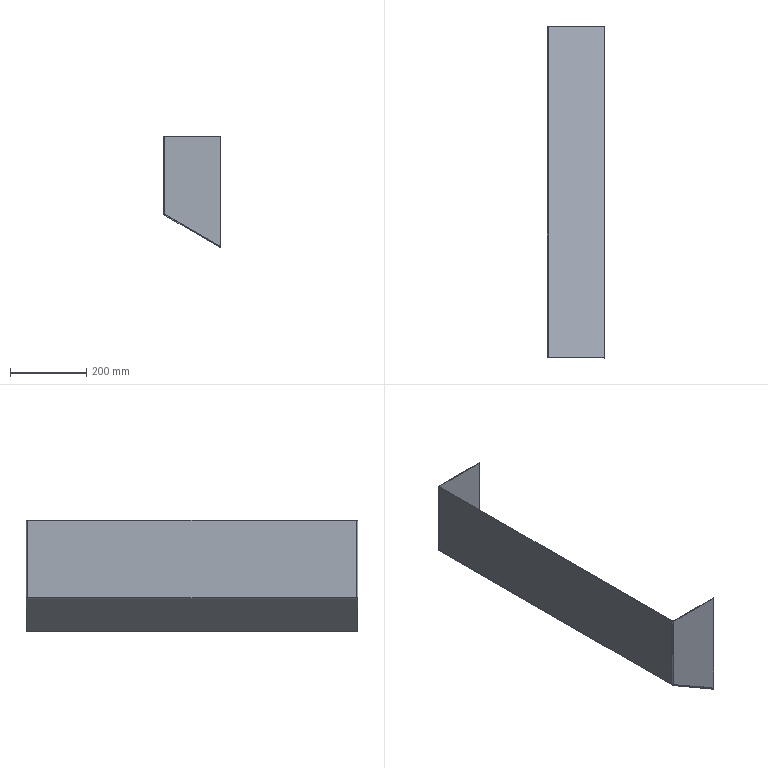Component | SolidWorks | AirInletUpperBeamAssembly-1_AirInletUpperBeamBaffle-2 | 1 solid | 32 faces | box 152 x 870 x 291.73 mm | volume 803027 mm3 | plane 24 | cylinder 6 | spline 2 | commonest cylinder face diameters 4 x3 8 x3 | material Plain Carbon Steel
STEP:
#1=COLOUR_RGB('',0.7922,0.8196,0.9333);
#2=FILL_AREA_STYLE_COLOUR('',#1);
#3=FILL_AREA_STYLE('',(#2));
#4=SURFACE_STYLE_FILL_AREA(#3);
#5=SURFACE_SIDE_STYLE('',(#4));
#6=SURFACE_STYLE_USAGE(.BOTH.,#5);
#7=PRESENTATION_STYLE_ASSIGNMENT((#6));
#8=CARTESIAN_POINT('',(95.562,7.226,69.616));
#9=VERTEX_POINT('',#8);
#10=CARTESIAN_POINT('',(95.562,41.163,69.616));
#11=VERTEX_POINT('',#10);
#12=CARTESIAN_POINT('',(95.562,7.069,69.616));
#13=DIRECTION('',(-0.,1.,-0.));
#14=VECTOR('',#13,39.37);
#15=LINE('',#12,#14);
#16=EDGE_CURVE('',#9,#11,#15,.T.);
#17=ORIENTED_EDGE('',*,*,#16,.T.);
#18=CARTESIAN_POINT('',(95.562,41.163,77.578));
#19=VERTEX_POINT('',#18);
#20=CARTESIAN_POINT('',(95.562,41.163,77.578));
#21=DIRECTION('',(0.,-0.,-1.));
#22=VECTOR('',#21,39.37);
#23=LINE('',#20,#22);
#24=EDGE_CURVE('',#19,#11,#23,.T.);
#25=ORIENTED_EDGE('',*,*,#24,.F.);
#26=CARTESIAN_POINT('',(95.562,7.226,77.578));
#27=VERTEX_POINT('',#26);
#28=CARTESIAN_POINT('',(95.562,7.069,77.578));
#29=DIRECTION('',(-0.,1.,-0.));
#30=VECTOR('',#29,39.37);
#31=LINE('',#28,#30);
#32=EDGE_CURVE('',#27,#19,#31,.T.);
#33=ORIENTED_EDGE('',*,*,#32,.F.);
#34=CARTESIAN_POINT('',(95.562,7.226,69.57));
#35=DIRECTION('',(-0.,0.,1.));
#36=VECTOR('',#35,39.37);
#37=LINE('',#34,#36);
#38=EDGE_CURVE('',#9,#27,#37,.T.);
#39=ORIENTED_EDGE('',*,*,#38,.F.);
#40=EDGE_LOOP('',(#17,#25,#33,#39));
#41=FACE_OUTER_BOUND('',#40,.T.);
#42=CARTESIAN_POINT('',(95.562,7.069,69.57));
#43=DIRECTION('',(1.,0.,-0.));
#44=DIRECTION('',(0.,0.,1.));
#45=AXIS2_PLACEMENT_3D('',#42,#43,#44);
#46=PLANE('',#45);
#47=ADVANCED_FACE('',(#41),#46,.T.);
#48=CARTESIAN_POINT('',(95.484,41.163,77.578));
#49=VERTEX_POINT('',#48);
#50=CARTESIAN_POINT('',(95.484,41.163,69.616));
#51=VERTEX_POINT('',#50);
#52=CARTESIAN_POINT('',(95.484,41.163,77.578));
#53=DIRECTION('',(0.,-0.,-1.));
#54=VECTOR('',#53,39.37);
#55=LINE('',#52,#54);
#56=EDGE_CURVE('',#49,#51,#55,.T.);
#57=ORIENTED_EDGE('',*,*,#56,.T.);
#58=CARTESIAN_POINT('',(95.484,7.226,69.616));
#59=VERTEX_POINT('',#58);
#60=CARTESIAN_POINT('',(95.484,7.069,69.616));
#61=DIRECTION('',(-0.,1.,-0.));
#62=VECTOR('',#61,39.37);
#63=LINE('',#60,#62);
#64=EDGE_CURVE('',#59,#51,#63,.T.);
#65=ORIENTED_EDGE('',*,*,#64,.F.);
#66=CARTESIAN_POINT('',(95.484,7.226,77.578));
#67=VERTEX_POINT('',#66);
#68=CARTESIAN_POINT('',(95.484,7.226,69.57));
#69=DIRECTION('',(-0.,0.,1.));
#70=VECTOR('',#69,39.37);
#71=LINE('',#68,#70);
#72=EDGE_CURVE('',#59,#67,#71,.T.);
#73=ORIENTED_EDGE('',*,*,#72,.T.);
#74=CARTESIAN_POINT('',(95.484,7.069,77.578));
#75=DIRECTION('',(-0.,1.,-0.));
#76=VECTOR('',#75,39.37);
#77=LINE('',#74,#76);
#78=EDGE_CURVE('',#67,#49,#77,.T.);
#79=ORIENTED_EDGE('',*,*,#78,.T.);
#80=EDGE_LOOP('',(#57,#65,#73,#79));
#81=FACE_OUTER_BOUND('',#80,.T.);
#82=CARTESIAN_POINT('',(95.484,7.069,69.57));
#83=DIRECTION('',(1.,0.,-0.));
#84=DIRECTION('',(0.,0.,1.));
#85=AXIS2_PLACEMENT_3D('',#82,#83,#84);
#86=PLANE('',#85);
#87=ADVANCED_FACE('',(#81),#86,.F.);
#88=ORIENTED_EDGE('',*,*,#32,.T.);
#89=CARTESIAN_POINT('',(95.562,41.163,77.578));
#90=DIRECTION('',(-1.,-0.,0.));
#91=VECTOR('',#90,39.37);
#92=LINE('',#89,#91);
#93=EDGE_CURVE('',#19,#49,#92,.T.);
#94=ORIENTED_EDGE('',*,*,#93,.T.);
#95=ORIENTED_EDGE('',*,*,#78,.F.);
#96=CARTESIAN_POINT('',(95.562,7.226,77.578));
#97=DIRECTION('',(-1.,-0.,0.));
#98=VECTOR('',#97,39.37);
#99=LINE('',#96,#98);
#100=EDGE_CURVE('',#27,#67,#99,.T.);
#101=ORIENTED_EDGE('',*,*,#100,.F.);
#102=EDGE_LOOP('',(#88,#94,#95,#101));
#103=FACE_OUTER_BOUND('',#102,.T.);
#104=CARTESIAN_POINT('',(95.484,7.069,77.578));
#105=DIRECTION('',(-0.,0.,1.));
#106=DIRECTION('',(0.,-1.,0.));
#107=AXIS2_PLACEMENT_3D('',#104,#105,#106);
#108=PLANE('',#107);
#109=ADVANCED_FACE('',(#103),#108,.T.);
#110=CARTESIAN_POINT('',(95.602,7.069,69.547));
#111=VERTEX_POINT('',#110);
#112=CARTESIAN_POINT('',(95.562,7.069,69.479));
#113=VERTEX_POINT('',#112);
#114=CARTESIAN_POINT('',(95.602,7.069,69.547));
#115=DIRECTION('',(-0.5,-0.,-0.866));
#116=VECTOR('',#115,39.37);
#117=LINE('',#114,#116);
#118=EDGE_CURVE('',#111,#113,#117,.T.);
#119=ORIENTED_EDGE('',*,*,#118,.F.);
#120=CARTESIAN_POINT('',(95.562,7.069,69.616));
#121=VERTEX_POINT('',#120);
#122=CARTESIAN_POINT('',(95.641,7.069,69.616));
#123=DIRECTION('',(0.,-1.,0.));
#124=DIRECTION('',(-1.,0.,0.));
#125=AXIS2_PLACEMENT_3D('',#122,#123,#124);
#126=CIRCLE('',#125,0.07874);
#127=EDGE_CURVE('',#121,#111,#126,.T.);
#128=ORIENTED_EDGE('',*,*,#127,.F.);
#129=CARTESIAN_POINT('',(95.484,7.069,69.616));
#130=VERTEX_POINT('',#129);
#131=CARTESIAN_POINT('',(95.484,7.069,69.616));
#132=DIRECTION('',(1.,0.,-0.));
#133=VECTOR('',#132,39.37);
#134=LINE('',#131,#133);
#135=EDGE_CURVE('',#130,#121,#134,.T.);
#136=ORIENTED_EDGE('',*,*,#135,.F.);
#137=CARTESIAN_POINT('',(95.641,7.069,69.616));
#138=DIRECTION('',(0.,-1.,0.));
#139=DIRECTION('',(1.,0.,0.));
#140=AXIS2_PLACEMENT_3D('',#137,#138,#139);
#141=CIRCLE('',#140,0.1575);
#142=EDGE_CURVE('',#130,#113,#141,.T.);
#143=ORIENTED_EDGE('',*,*,#142,.T.);
#144=EDGE_LOOP('',(#119,#128,#136,#143));
#145=FACE_OUTER_BOUND('',#144,.T.);
#146=CARTESIAN_POINT('',(95.602,7.069,69.547));
#147=DIRECTION('',(0.,-1.,0.));
#148=DIRECTION('',(1.,0.,-0.));
#149=AXIS2_PLACEMENT_3D('',#146,#147,#148);
#150=PLANE('',#149);
#151=ADVANCED_FACE('',(#145),#150,.T.);
#152=CARTESIAN_POINT('',(101.468,7.069,66.161));
#153=VERTEX_POINT('',#152);
#154=CARTESIAN_POINT('',(95.562,7.069,69.57));
#155=DIRECTION('',(0.866,0.,-0.5));
#156=VECTOR('',#155,39.37);
#157=LINE('',#154,#156);
#158=EDGE_CURVE('',#111,#153,#157,.T.);
#159=ORIENTED_EDGE('',*,*,#158,.F.);
#160=ORIENTED_EDGE('',*,*,#118,.T.);
#161=CARTESIAN_POINT('',(101.429,7.069,66.092));
#162=VERTEX_POINT('',#161);
#163=CARTESIAN_POINT('',(95.523,7.069,69.502));
#164=DIRECTION('',(0.866,0.,-0.5));
#165=VECTOR('',#164,39.37);
#166=LINE('',#163,#165);
#167=EDGE_CURVE('',#113,#162,#166,.T.);
#168=ORIENTED_EDGE('',*,*,#167,.T.);
#169=CARTESIAN_POINT('',(101.468,7.069,66.161));
#170=DIRECTION('',(-0.5,-0.,-0.866));
#171=VECTOR('',#170,39.37);
#172=LINE('',#169,#171);
#173=EDGE_CURVE('',#153,#162,#172,.T.);
#174=ORIENTED_EDGE('',*,*,#173,.F.);
#175=EDGE_LOOP('',(#159,#160,#168,#174));
#176=FACE_OUTER_BOUND('',#175,.T.);
#177=CARTESIAN_POINT('',(95.484,7.069,69.616));
#178=DIRECTION('',(0.,-1.,0.));
#179=DIRECTION('',(1.,0.,-0.));
#180=AXIS2_PLACEMENT_3D('',#177,#178,#179);
#181=PLANE('',#180);
#182=ADVANCED_FACE('',(#176),#181,.T.);
#183=CARTESIAN_POINT('',(95.562,41.321,69.616));
#184=VERTEX_POINT('',#183);
#185=CARTESIAN_POINT('',(95.484,41.321,69.616));
#186=VERTEX_POINT('',#185);
#187=CARTESIAN_POINT('',(95.562,41.321,69.616));
#188=DIRECTION('',(-1.,-0.,0.));
#189=VECTOR('',#188,39.37);
#190=LINE('',#187,#189);
#191=EDGE_CURVE('',#184,#186,#190,.T.);
#192=ORIENTED_EDGE('',*,*,#191,.F.);
#193=CARTESIAN_POINT('',(95.602,41.321,69.547));
#194=VERTEX_POINT('',#193);
#195=CARTESIAN_POINT('',(95.641,41.321,69.616));
#196=DIRECTION('',(0.,-1.,0.));
#197=DIRECTION('',(-1.,0.,0.));
#198=AXIS2_PLACEMENT_3D('',#195,#196,#197);
#199=CIRCLE('',#198,0.07874);
#200=EDGE_CURVE('',#184,#194,#199,.T.);
#201=ORIENTED_EDGE('',*,*,#200,.T.);
#202=CARTESIAN_POINT('',(95.562,41.321,69.479));
#203=VERTEX_POINT('',#202);
#204=CARTESIAN_POINT('',(95.562,41.321,69.479));
#205=DIRECTION('',(0.5,0.,0.866));
#206=VECTOR('',#205,39.37);
#207=LINE('',#204,#206);
#208=EDGE_CURVE('',#203,#194,#207,.T.);
#209=ORIENTED_EDGE('',*,*,#208,.F.);
#210=CARTESIAN_POINT('',(95.641,41.321,69.616));
#211=DIRECTION('',(0.,-1.,0.));
#212=DIRECTION('',(1.,0.,0.));
#213=AXIS2_PLACEMENT_3D('',#210,#211,#212);
#214=CIRCLE('',#213,0.1575);
#215=EDGE_CURVE('',#186,#203,#214,.T.);
#216=ORIENTED_EDGE('',*,*,#215,.F.);
#217=EDGE_LOOP('',(#192,#201,#209,#216));
#218=FACE_OUTER_BOUND('',#217,.T.);
#219=CARTESIAN_POINT('',(95.562,41.321,69.616));
#220=DIRECTION('',(-0.,1.,-0.));
#221=DIRECTION('',(-1.,-0.,0.));
#222=AXIS2_PLACEMENT_3D('',#219,#220,#221);
#223=PLANE('',#222);
#224=ADVANCED_FACE('',(#218),#223,.T.);
#225=CARTESIAN_POINT('',(101.429,41.321,66.092));
#226=VERTEX_POINT('',#225);
#227=CARTESIAN_POINT('',(95.523,41.321,69.502));
#228=DIRECTION('',(0.866,0.,-0.5));
#229=VECTOR('',#228,39.37);
#230=LINE('',#227,#229);
#231=EDGE_CURVE('',#203,#226,#230,.T.);
#232=ORIENTED_EDGE('',*,*,#231,.T.);
#233=CARTESIAN_POINT('',(101.429,7.069,66.092));
#234=DIRECTION('',(-0.,1.,-0.));
#235=VECTOR('',#234,39.37);
#236=LINE('',#233,#235);
#237=EDGE_CURVE('',#162,#226,#236,.T.);
#238=ORIENTED_EDGE('',*,*,#237,.F.);
#239=ORIENTED_EDGE('',*,*,#167,.F.);
#240=CARTESIAN_POINT('',(95.562,7.069,69.479));
#241=DIRECTION('',(-0.,1.,-0.));
#242=VECTOR('',#241,39.37);
#243=LINE('',#240,#242);
#244=EDGE_CURVE('',#113,#203,#243,.T.);
#245=ORIENTED_EDGE('',*,*,#244,.T.);
#246=EDGE_LOOP('',(#232,#238,#239,#245));
#247=FACE_OUTER_BOUND('',#246,.T.);
#248=CARTESIAN_POINT('',(95.523,7.069,69.502));
#249=DIRECTION('',(0.5,0.,0.866));
#250=DIRECTION('',(-0.866,-0.,0.5));
#251=AXIS2_PLACEMENT_3D('',#248,#249,#250);
#252=PLANE('',#251);
#253=ADVANCED_FACE('',(#247),#252,.F.);
#254=CARTESIAN_POINT('',(101.468,41.321,66.161));
#255=VERTEX_POINT('',#254);
#256=CARTESIAN_POINT('',(101.468,41.321,66.161));
#257=DIRECTION('',(-0.5,-0.,-0.866));
#258=VECTOR('',#257,39.37);
#259=LINE('',#256,#258);
#260=EDGE_CURVE('',#255,#226,#259,.T.);
#261=ORIENTED_EDGE('',*,*,#260,.F.);
#262=CARTESIAN_POINT('',(101.468,7.069,66.161));
#263=DIRECTION('',(-0.,1.,-0.));
#264=VECTOR('',#263,39.37);
#265=LINE('',#262,#264);
#266=EDGE_CURVE('',#153,#255,#265,.T.);
#267=ORIENTED_EDGE('',*,*,#266,.F.);
#268=ORIENTED_EDGE('',*,*,#173,.T.);
#269=ORIENTED_EDGE('',*,*,#237,.T.);
#270=EDGE_LOOP('',(#261,#267,#268,#269));
#271=FACE_OUTER_BOUND('',#270,.T.);
#272=CARTESIAN_POINT('',(101.468,7.069,66.161));
#273=DIRECTION('',(0.866,0.,-0.5));
#274=DIRECTION('',(0.5,0.,0.866));
#275=AXIS2_PLACEMENT_3D('',#272,#273,#274);
#276=PLANE('',#275);
#277=ADVANCED_FACE('',(#271),#276,.T.);
#278=CARTESIAN_POINT('',(95.562,41.321,69.57));
#279=DIRECTION('',(0.866,0.,-0.5));
#280=VECTOR('',#279,39.37);
#281=LINE('',#278,#280);
#282=EDGE_CURVE('',#194,#255,#281,.T.);
#283=ORIENTED_EDGE('',*,*,#282,.F.);
#284=CARTESIAN_POINT('',(95.602,7.069,69.547));
#285=DIRECTION('',(-0.,1.,-0.));
#286=VECTOR('',#285,39.37);
#287=LINE('',#284,#286);
#288=EDGE_CURVE('',#111,#194,#287,.T.);
#289=ORIENTED_EDGE('',*,*,#288,.F.);
#290=ORIENTED_EDGE('',*,*,#158,.T.);
#291=ORIENTED_EDGE('',*,*,#266,.T.);
#292=EDGE_LOOP('',(#283,#289,#290,#291));
#293=FACE_OUTER_BOUND('',#292,.T.);
#294=CARTESIAN_POINT('',(95.562,7.069,69.57));
#295=DIRECTION('',(0.5,0.,0.866));
#296=DIRECTION('',(-0.866,-0.,0.5));
#297=AXIS2_PLACEMENT_3D('',#294,#295,#296);
#298=PLANE('',#297);
#299=ADVANCED_FACE('',(#293),#298,.T.);
#300=ORIENTED_EDGE('',*,*,#200,.F.);
#301=CARTESIAN_POINT('',(95.562,41.163,69.616));
#302=DIRECTION('',(-0.,1.,0.));
#303=VECTOR('',#302,39.37);
#304=LINE('',#301,#303);
#305=EDGE_CURVE('',#11,#184,#304,.T.);
#306=ORIENTED_EDGE('',*,*,#305,.F.);
#307=ORIENTED_EDGE('',*,*,#16,.F.);
#308=CARTESIAN_POINT('',(95.562,7.069,69.616));
#309=DIRECTION('',(-0.,1.,-0.));
#310=VECTOR('',#309,39.37);
#311=LINE('',#308,#310);
#312=EDGE_CURVE('',#121,#9,#311,.T.);
#313=ORIENTED_EDGE('',*,*,#312,.F.);
#314=ORIENTED_EDGE('',*,*,#127,.T.);
#315=ORIENTED_EDGE('',*,*,#288,.T.);
#316=EDGE_LOOP('',(#300,#306,#307,#313,#314,#315));
#317=FACE_OUTER_BOUND('',#316,.T.);
#318=CARTESIAN_POINT('',(95.641,7.069,69.616));
#319=DIRECTION('',(-0.,1.,-0.));
#320=DIRECTION('',(-1.,0.,0.));
#321=AXIS2_PLACEMENT_3D('',#318,#319,#320);
#322=CYLINDRICAL_SURFACE('',#321,0.07874);
#323=ADVANCED_FACE('',(#317),#322,.F.);
#324=ORIENTED_EDGE('',*,*,#215,.T.);
#325=ORIENTED_EDGE('',*,*,#244,.F.);
#326=ORIENTED_EDGE('',*,*,#142,.F.);
#327=CARTESIAN_POINT('',(95.484,7.069,69.616));
#328=DIRECTION('',(-0.,1.,-0.));
#329=VECTOR('',#328,39.37);
#330=LINE('',#327,#329);
#331=EDGE_CURVE('',#130,#59,#330,.T.);
#332=ORIENTED_EDGE('',*,*,#331,.T.);
#333=ORIENTED_EDGE('',*,*,#64,.T.);
#334=CARTESIAN_POINT('',(95.484,7.069,69.616));
#335=DIRECTION('',(-0.,1.,-0.));
#336=VECTOR('',#335,39.37);
#337=LINE('',#334,#336);
#338=EDGE_CURVE('',#51,#186,#337,.T.);
#339=ORIENTED_EDGE('',*,*,#338,.T.);
#340=EDGE_LOOP('',(#324,#325,#326,#332,#333,#339));
#341=FACE_OUTER_BOUND('',#340,.T.);
#342=CARTESIAN_POINT('',(95.641,7.069,69.616));
#343=DIRECTION('',(-0.,1.,-0.));
#344=DIRECTION('',(-1.,-0.,0.));
#345=AXIS2_PLACEMENT_3D('',#342,#343,#344);
#346=CYLINDRICAL_SURFACE('',#345,0.1575);
#347=ADVANCED_FACE('',(#341),#346,.T.);
#348=ORIENTED_EDGE('',*,*,#231,.F.);
#349=ORIENTED_EDGE('',*,*,#208,.T.);
#350=ORIENTED_EDGE('',*,*,#282,.T.);
#351=ORIENTED_EDGE('',*,*,#260,.T.);
#352=EDGE_LOOP('',(#348,#349,#350,#351));
#353=FACE_OUTER_BOUND('',#352,.T.);
#354=CARTESIAN_POINT('',(95.641,41.321,69.616));
#355=DIRECTION('',(-0.,1.,-0.));
#356=DIRECTION('',(-1.,-0.,0.));
#357=AXIS2_PLACEMENT_3D('',#354,#355,#356);
#358=PLANE('',#357);
#359=ADVANCED_FACE('',(#353),#358,.T.);
#360=CARTESIAN_POINT('',(95.562,7.226,69.616));
#361=DIRECTION('',(-1.,-0.,0.));
#362=VECTOR('',#361,39.37);
#363=LINE('',#360,#362);
#364=EDGE_CURVE('',#9,#59,#363,.T.);
#365=ORIENTED_EDGE('',*,*,#364,.T.);
#366=ORIENTED_EDGE('',*,*,#331,.F.);
#367=ORIENTED_EDGE('',*,*,#135,.T.);
#368=ORIENTED_EDGE('',*,*,#312,.T.);
#369=EDGE_LOOP('',(#365,#366,#367,#368));
#370=FACE_OUTER_BOUND('',#369,.T.);
#371=CARTESIAN_POINT('',(95.562,7.069,69.616));
#372=DIRECTION('',(0.,0.,1.));
#373=DIRECTION('',(0.,-1.,0.));
#374=AXIS2_PLACEMENT_3D('',#371,#372,#373);
#375=PLANE('',#374);
#376=ADVANCED_FACE('',(#370),#375,.T.);
#377=CARTESIAN_POINT('',(95.641,7.148,77.578));
#378=VERTEX_POINT('',#377);
#379=CARTESIAN_POINT('',(95.641,7.069,77.578));
#380=VERTEX_POINT('',#379);
#381=CARTESIAN_POINT('',(95.641,7.069,77.578));
#382=DIRECTION('',(0.,-1.,0.));
#383=VECTOR('',#382,39.37);
#384=LINE('',#381,#383);
#385=EDGE_CURVE('',#378,#380,#384,.T.);
#386=ORIENTED_EDGE('',*,*,#385,.F.);
#387=CARTESIAN_POINT('',(95.641,7.226,77.578));
#388=DIRECTION('',(-0.,0.,1.));
#389=DIRECTION('',(0.,1.,0.));
#390=AXIS2_PLACEMENT_3D('',#387,#388,#389);
#391=CIRCLE('',#390,0.07874);
#392=EDGE_CURVE('',#27,#378,#391,.T.);
#393=ORIENTED_EDGE('',*,*,#392,.F.);
#394=ORIENTED_EDGE('',*,*,#100,.T.);
#395=CARTESIAN_POINT('',(95.641,7.226,77.578));
#396=DIRECTION('',(-0.,0.,1.));
#397=DIRECTION('',(0.,1.,0.));
#398=AXIS2_PLACEMENT_3D('',#395,#396,#397);
#399=CIRCLE('',#398,0.1575);
#400=EDGE_CURVE('',#67,#380,#399,.T.);
#401=ORIENTED_EDGE('',*,*,#400,.T.);
#402=EDGE_LOOP('',(#386,#393,#394,#401));
#403=FACE_OUTER_BOUND('',#402,.T.);
#404=CARTESIAN_POINT('',(95.641,7.226,77.578));
#405=DIRECTION('',(-0.,0.,1.));
#406=DIRECTION('',(0.,-1.,0.));
#407=AXIS2_PLACEMENT_3D('',#404,#405,#406);
#408=PLANE('',#407);
#409=ADVANCED_FACE('',(#403),#408,.T.);
#410=CARTESIAN_POINT('',(95.641,7.148,69.57));
#411=VERTEX_POINT('',#410);
#412=CARTESIAN_POINT('',(95.641,7.148,69.57));
#413=CARTESIAN_POINT('',(95.636,7.148,69.572));
#414=CARTESIAN_POINT('',(95.631,7.148,69.574));
#415=CARTESIAN_POINT('',(95.621,7.15,69.578));
#416=CARTESIAN_POINT('',(95.616,7.152,69.58));
#417=CARTESIAN_POINT('',(95.606,7.156,69.583));
#418=CARTESIAN_POINT('',(95.602,7.158,69.585));
#419=CARTESIAN_POINT('',(95.593,7.164,69.589));
#420=CARTESIAN_POINT('',(95.589,7.167,69.591));
#421=CARTESIAN_POINT('',(95.582,7.174,69.595));
#422=CARTESIAN_POINT('',(95.579,7.178,69.597));
#423=CARTESIAN_POINT('',(95.573,7.187,69.6));
#424=CARTESIAN_POINT('',(95.57,7.191,69.602));
#425=CARTESIAN_POINT('',(95.567,7.201,69.606));
#426=CARTESIAN_POINT('',(95.565,7.206,69.608));
#427=CARTESIAN_POINT('',(95.563,7.216,69.612));
#428=CARTESIAN_POINT('',(95.562,7.221,69.614));
#429=CARTESIAN_POINT('',(95.562,7.226,69.616));
#430=B_SPLINE_CURVE_WITH_KNOTS('',3,(#412,#413,#414,#415,#416,#417,#418,#419,#420,#421,#422,#423,#424,#425,#426,#427,#428,#429),.UNSPECIFIED.,.F.,.F.,(4,2,2,2,2,2,2,2,4),(0.,0.0004161,0.0008322,0.001248,0.001664,0.002081,0.002497,0.002913,0.003329),.UNSPECIFIED.);
#431=EDGE_CURVE('',#411,#9,#430,.T.);
#432=ORIENTED_EDGE('',*,*,#431,.F.);
#433=CARTESIAN_POINT('',(95.641,7.069,69.57));
#434=VERTEX_POINT('',#433);
#435=CARTESIAN_POINT('',(95.641,7.148,69.57));
#436=DIRECTION('',(0.,-1.,-0.));
#437=VECTOR('',#436,39.37);
#438=LINE('',#435,#437);
#439=EDGE_CURVE('',#411,#434,#438,.T.);
#440=ORIENTED_EDGE('',*,*,#439,.T.);
#441=CARTESIAN_POINT('',(95.641,7.069,69.57));
#442=CARTESIAN_POINT('',(95.631,7.069,69.572));
#443=CARTESIAN_POINT('',(95.621,7.07,69.574));
#444=CARTESIAN_POINT('',(95.6,7.074,69.578));
#445=CARTESIAN_POINT('',(95.59,7.077,69.58));
#446=CARTESIAN_POINT('',(95.571,7.085,69.583));
#447=CARTESIAN_POINT('',(95.562,7.09,69.585));
#448=CARTESIAN_POINT('',(95.545,7.101,69.589));
#449=CARTESIAN_POINT('',(95.537,7.108,69.591));
#450=CARTESIAN_POINT('',(95.523,7.122,69.595));
#451=CARTESIAN_POINT('',(95.516,7.13,69.597));
#452=CARTESIAN_POINT('',(95.505,7.147,69.6));
#453=CARTESIAN_POINT('',(95.5,7.156,69.602));
#454=CARTESIAN_POINT('',(95.488,7.185,69.608));
#455=CARTESIAN_POINT('',(95.484,7.206,69.612));
#456=CARTESIAN_POINT('',(95.484,7.226,69.616));
#457=B_SPLINE_CURVE_WITH_KNOTS('',3,(#441,#442,#443,#444,#445,#446,#447,#448,#449,#450,#451,#452,#453,#454,#455,#456),.UNSPECIFIED.,.F.,.F.,(4,2,2,2,2,2,2,4),(0.,0.0007941,0.001588,0.002382,0.003177,0.003971,0.004765,0.006353),.UNSPECIFIED.);
#458=EDGE_CURVE('',#434,#59,#457,.T.);
#459=ORIENTED_EDGE('',*,*,#458,.T.);
#460=ORIENTED_EDGE('',*,*,#364,.F.);
#461=EDGE_LOOP('',(#432,#440,#459,#460));
#462=FACE_OUTER_BOUND('',#461,.T.);
#463=CARTESIAN_POINT('',(95.641,7.068,69.57));
#464=CARTESIAN_POINT('',(95.62,7.068,69.574));
#465=CARTESIAN_POINT('',(95.6,7.072,69.578));
#466=CARTESIAN_POINT('',(95.562,7.088,69.585));
#467=CARTESIAN_POINT('',(95.544,7.1,69.589));
#468=CARTESIAN_POINT('',(95.515,7.129,69.597));
#469=CARTESIAN_POINT('',(95.503,7.147,69.6));
#470=CARTESIAN_POINT('',(95.487,7.185,69.608));
#471=CARTESIAN_POINT('',(95.483,7.206,69.612));
#472=CARTESIAN_POINT('',(95.483,7.226,69.616));
#473=CARTESIAN_POINT('',(95.641,7.069,69.57));
#474=CARTESIAN_POINT('',(95.621,7.069,69.574));
#475=CARTESIAN_POINT('',(95.6,7.073,69.578));
#476=CARTESIAN_POINT('',(95.562,7.089,69.585));
#477=CARTESIAN_POINT('',(95.544,7.1,69.589));
#478=CARTESIAN_POINT('',(95.515,7.13,69.597));
#479=CARTESIAN_POINT('',(95.504,7.147,69.6));
#480=CARTESIAN_POINT('',(95.488,7.185,69.608));
#481=CARTESIAN_POINT('',(95.484,7.206,69.612));
#482=CARTESIAN_POINT('',(95.484,7.226,69.616));
#483=CARTESIAN_POINT('',(95.641,7.148,69.57));
#484=CARTESIAN_POINT('',(95.631,7.148,69.574));
#485=CARTESIAN_POINT('',(95.621,7.15,69.578));
#486=CARTESIAN_POINT('',(95.602,7.158,69.585));
#487=CARTESIAN_POINT('',(95.593,7.163,69.589));
#488=CARTESIAN_POINT('',(95.578,7.178,69.597));
#489=CARTESIAN_POINT('',(95.572,7.187,69.6));
#490=CARTESIAN_POINT('',(95.565,7.206,69.608));
#491=CARTESIAN_POINT('',(95.562,7.216,69.612));
#492=CARTESIAN_POINT('',(95.562,7.226,69.616));
#493=CARTESIAN_POINT('',(95.641,7.148,69.57));
#494=CARTESIAN_POINT('',(95.631,7.148,69.574));
#495=CARTESIAN_POINT('',(95.621,7.15,69.578));
#496=CARTESIAN_POINT('',(95.602,7.158,69.585));
#497=CARTESIAN_POINT('',(95.593,7.164,69.589));
#498=CARTESIAN_POINT('',(95.579,7.178,69.597));
#499=CARTESIAN_POINT('',(95.573,7.187,69.6));
#500=CARTESIAN_POINT('',(95.565,7.206,69.608));
#501=CARTESIAN_POINT('',(95.563,7.216,69.612));
#502=CARTESIAN_POINT('',(95.563,7.226,69.616));
#503=B_SPLINE_SURFACE_WITH_KNOTS('',1,3,((#463,#464,#465,#466,#467,#468,#469,#470,#471,#472),(#473,#474,#475,#476,#477,#478,#479,#480,#481,#482),(#483,#484,#485,#486,#487,#488,#489,#490,#491,#492),(#493,#494,#495,#496,#497,#498,#499,#500,#501,#502)),.UNSPECIFIED.,.F.,.F.,.F.,(2,1,1,2),(4,2,2,2,4),(-0.01,0.,1.,1.01),(0.,0.25,0.5,0.75,1.),.UNSPECIFIED.);
#504=ADVANCED_FACE('',(#462),#503,.F.);
#505=ORIENTED_EDGE('',*,*,#72,.F.);
#506=ORIENTED_EDGE('',*,*,#458,.F.);
#507=CARTESIAN_POINT('',(95.641,7.069,77.578));
#508=DIRECTION('',(-0.,0.,1.));
#509=VECTOR('',#508,39.37);
#510=LINE('',#507,#509);
#511=EDGE_CURVE('',#434,#380,#510,.T.);
#512=ORIENTED_EDGE('',*,*,#511,.T.);
#513=ORIENTED_EDGE('',*,*,#400,.F.);
#514=EDGE_LOOP('',(#505,#506,#512,#513));
#515=FACE_OUTER_BOUND('',#514,.T.);
#516=CARTESIAN_POINT('',(95.641,7.226,69.57));
#517=DIRECTION('',(0.,-0.,-1.));
#518=DIRECTION('',(0.,-1.,0.));
#519=AXIS2_PLACEMENT_3D('',#516,#517,#518);
#520=CYLINDRICAL_SURFACE('',#519,0.1575);
#521=ADVANCED_FACE('',(#515),#520,.T.);
#522=ORIENTED_EDGE('',*,*,#38,.T.);
#523=ORIENTED_EDGE('',*,*,#392,.T.);
#524=CARTESIAN_POINT('',(95.641,7.148,77.578));
#525=DIRECTION('',(0.,-0.,-1.));
#526=VECTOR('',#525,39.37);
#527=LINE('',#524,#526);
#528=EDGE_CURVE('',#378,#411,#527,.T.);
#529=ORIENTED_EDGE('',*,*,#528,.T.);
#530=ORIENTED_EDGE('',*,*,#431,.T.);
#531=EDGE_LOOP('',(#522,#523,#529,#530));
#532=FACE_OUTER_BOUND('',#531,.T.);
#533=CARTESIAN_POINT('',(95.641,7.226,69.57));
#534=DIRECTION('',(0.,-0.,-1.));
#535=DIRECTION('',(0.,-1.,0.));
#536=AXIS2_PLACEMENT_3D('',#533,#534,#535);
#537=CYLINDRICAL_SURFACE('',#536,0.07874);
#538=ADVANCED_FACE('',(#532),#537,.F.);
#539=ORIENTED_EDGE('',*,*,#385,.T.);
#540=CARTESIAN_POINT('',(101.468,7.069,77.578));
#541=VERTEX_POINT('',#540);
#542=CARTESIAN_POINT('',(95.562,7.069,77.578));
#543=DIRECTION('',(-1.,0.,0.));
#544=VECTOR('',#543,39.37);
#545=LINE('',#542,#544);
#546=EDGE_CURVE('',#541,#380,#545,.T.);
#547=ORIENTED_EDGE('',*,*,#546,.F.);
#548=CARTESIAN_POINT('',(101.468,7.148,77.578));
#549=VERTEX_POINT('',#548);
#550=CARTESIAN_POINT('',(101.468,7.069,77.578));
#551=DIRECTION('',(-0.,1.,-0.));
#552=VECTOR('',#551,39.37);
#553=LINE('',#550,#552);
#554=EDGE_CURVE('',#541,#549,#553,.T.);
#555=ORIENTED_EDGE('',*,*,#554,.T.);
#556=CARTESIAN_POINT('',(95.562,7.148,77.578));
#557=DIRECTION('',(-1.,0.,0.));
#558=VECTOR('',#557,39.37);
#559=LINE('',#556,#558);
#560=EDGE_CURVE('',#549,#378,#559,.T.);
#561=ORIENTED_EDGE('',*,*,#560,.T.);
#562=EDGE_LOOP('',(#539,#547,#555,#561));
#563=FACE_OUTER_BOUND('',#562,.T.);
#564=CARTESIAN_POINT('',(95.562,7.069,77.578));
#565=DIRECTION('',(0.,-0.,-1.));
#566=DIRECTION('',(-0.,1.,-0.));
#567=AXIS2_PLACEMENT_3D('',#564,#565,#566);
#568=PLANE('',#567);
#569=ADVANCED_FACE('',(#563),#568,.F.);
#570=ORIENTED_EDGE('',*,*,#439,.F.);
#571=CARTESIAN_POINT('',(101.468,7.148,66.206));
#572=VERTEX_POINT('',#571);
#573=CARTESIAN_POINT('',(95.562,7.148,69.616));
#574=DIRECTION('',(0.866,-0.,-0.5));
#575=VECTOR('',#574,39.37);
#576=LINE('',#573,#575);
#577=EDGE_CURVE('',#411,#572,#576,.T.);
#578=ORIENTED_EDGE('',*,*,#577,.T.);
#579=CARTESIAN_POINT('',(101.468,7.069,66.206));
#580=VERTEX_POINT('',#579);
#581=CARTESIAN_POINT('',(101.468,7.069,66.206));
#582=DIRECTION('',(-0.,1.,-0.));
#583=VECTOR('',#582,39.37);
#584=LINE('',#581,#583);
#585=EDGE_CURVE('',#580,#572,#584,.T.);
#586=ORIENTED_EDGE('',*,*,#585,.F.);
#587=CARTESIAN_POINT('',(95.582,7.069,69.604));
#588=DIRECTION('',(0.866,-0.,-0.5));
#589=VECTOR('',#588,39.37);
#590=LINE('',#587,#589);
#591=EDGE_CURVE('',#434,#580,#590,.T.);
#592=ORIENTED_EDGE('',*,*,#591,.F.);
#593=EDGE_LOOP('',(#570,#578,#586,#592));
#594=FACE_OUTER_BOUND('',#593,.T.);
#595=CARTESIAN_POINT('',(95.562,7.069,69.616));
#596=DIRECTION('',(0.5,0.,0.866));
#597=DIRECTION('',(-0.866,-0.,0.5));
#598=AXIS2_PLACEMENT_3D('',#595,#596,#597);
#599=PLANE('',#598);
#600=ADVANCED_FACE('',(#594),#599,.F.);
#601=ORIENTED_EDGE('',*,*,#511,.F.);
#602=ORIENTED_EDGE('',*,*,#591,.T.);
#603=CARTESIAN_POINT('',(101.468,7.069,69.57));
#604=DIRECTION('',(-0.,0.,1.));
#605=VECTOR('',#604,39.37);
#606=LINE('',#603,#605);
#607=EDGE_CURVE('',#580,#541,#606,.T.);
#608=ORIENTED_EDGE('',*,*,#607,.T.);
#609=ORIENTED_EDGE('',*,*,#546,.T.);
#610=EDGE_LOOP('',(#601,#602,#608,#609));
#611=FACE_OUTER_BOUND('',#610,.T.);
#612=CARTESIAN_POINT('',(95.562,7.069,69.57));
#613=DIRECTION('',(0.,1.,-0.));
#614=DIRECTION('',(-1.,0.,0.));
#615=AXIS2_PLACEMENT_3D('',#612,#613,#614);
#616=PLANE('',#615);
#617=ADVANCED_FACE('',(#611),#616,.F.);
#618=ORIENTED_EDGE('',*,*,#577,.F.);
#619=ORIENTED_EDGE('',*,*,#528,.F.);
#620=ORIENTED_EDGE('',*,*,#560,.F.);
#621=CARTESIAN_POINT('',(101.468,7.148,77.578));
#622=DIRECTION('',(-0.,0.,1.));
#623=VECTOR('',#622,39.37);
#624=LINE('',#621,#623);
#625=EDGE_CURVE('',#572,#549,#624,.T.);
#626=ORIENTED_EDGE('',*,*,#625,.F.);
#627=EDGE_LOOP('',(#618,#619,#620,#626));
#628=FACE_OUTER_BOUND('',#627,.T.);
#629=CARTESIAN_POINT('',(95.562,7.148,69.57));
#630=DIRECTION('',(0.,1.,-0.));
#631=DIRECTION('',(-1.,0.,0.));
#632=AXIS2_PLACEMENT_3D('',#629,#630,#631);
#633=PLANE('',#632);
#634=ADVANCED_FACE('',(#628),#633,.T.);
#635=ORIENTED_EDGE('',*,*,#625,.T.);
#636=ORIENTED_EDGE('',*,*,#554,.F.);
#637=ORIENTED_EDGE('',*,*,#607,.F.);
#638=ORIENTED_EDGE('',*,*,#585,.T.);
#639=EDGE_LOOP('',(#635,#636,#637,#638));
#640=FACE_OUTER_BOUND('',#639,.T.);
#641=CARTESIAN_POINT('',(101.468,7.069,77.578));
#642=DIRECTION('',(-1.,-0.,0.));
#643=DIRECTION('',(0.,-1.,0.));
#644=AXIS2_PLACEMENT_3D('',#641,#642,#643);
#645=PLANE('',#644);
#646=ADVANCED_FACE('',(#640),#645,.F.);
#647=ORIENTED_EDGE('',*,*,#191,.T.);
#648=ORIENTED_EDGE('',*,*,#338,.F.);
#649=CARTESIAN_POINT('',(95.562,41.163,69.616));
#650=DIRECTION('',(-1.,-0.,0.));
#651=VECTOR('',#650,39.37);
#652=LINE('',#649,#651);
#653=EDGE_CURVE('',#11,#51,#652,.T.);
#654=ORIENTED_EDGE('',*,*,#653,.F.);
#655=ORIENTED_EDGE('',*,*,#305,.T.);
#656=EDGE_LOOP('',(#647,#648,#654,#655));
#657=FACE_OUTER_BOUND('',#656,.T.);
#658=CARTESIAN_POINT('',(95.562,41.163,69.616));
#659=DIRECTION('',(0.,-0.,1.));
#660=DIRECTION('',(0.,-1.,-0.));
#661=AXIS2_PLACEMENT_3D('',#658,#659,#660);
#662=PLANE('',#661);
#663=ADVANCED_FACE('',(#657),#662,.T.);
#664=CARTESIAN_POINT('',(95.641,41.242,69.57));
#665=VERTEX_POINT('',#664);
#666=CARTESIAN_POINT('',(95.641,41.321,69.57));
#667=VERTEX_POINT('',#666);
#668=CARTESIAN_POINT('',(95.641,41.321,69.57));
#669=DIRECTION('',(-0.,1.,-0.));
#670=VECTOR('',#669,39.37);
#671=LINE('',#668,#670);
#672=EDGE_CURVE('',#665,#667,#671,.T.);
#673=ORIENTED_EDGE('',*,*,#672,.F.);
#674=CARTESIAN_POINT('',(95.562,41.163,69.616));
#675=CARTESIAN_POINT('',(95.562,41.169,69.614));
#676=CARTESIAN_POINT('',(95.563,41.174,69.612));
#677=CARTESIAN_POINT('',(95.565,41.184,69.608));
#678=CARTESIAN_POINT('',(95.566,41.189,69.606));
#679=CARTESIAN_POINT('',(95.57,41.198,69.602));
#680=CARTESIAN_POINT('',(95.573,41.203,69.6));
#681=CARTESIAN_POINT('',(95.579,41.211,69.597));
#682=CARTESIAN_POINT('',(95.582,41.215,69.595));
#683=CARTESIAN_POINT('',(95.589,41.223,69.591));
#684=CARTESIAN_POINT('',(95.593,41.226,69.589));
#685=CARTESIAN_POINT('',(95.602,41.232,69.585));
#686=CARTESIAN_POINT('',(95.606,41.234,69.583));
#687=CARTESIAN_POINT('',(95.616,41.238,69.58));
#688=CARTESIAN_POINT('',(95.621,41.24,69.578));
#689=CARTESIAN_POINT('',(95.631,41.242,69.574));
#690=CARTESIAN_POINT('',(95.636,41.242,69.572));
#691=CARTESIAN_POINT('',(95.641,41.242,69.57));
#692=B_SPLINE_CURVE_WITH_KNOTS('',3,(#674,#675,#676,#677,#678,#679,#680,#681,#682,#683,#684,#685,#686,#687,#688,#689,#690,#691),.UNSPECIFIED.,.F.,.F.,(4,2,2,2,2,2,2,2,4),(0.,0.0004161,0.0008322,0.001248,0.001664,0.002081,0.002497,0.002913,0.003329),.UNSPECIFIED.);
#693=EDGE_CURVE('',#11,#665,#692,.T.);
#694=ORIENTED_EDGE('',*,*,#693,.F.);
#695=ORIENTED_EDGE('',*,*,#653,.T.);
#696=CARTESIAN_POINT('',(95.484,41.163,69.616));
#697=CARTESIAN_POINT('',(95.484,41.174,69.614));
#698=CARTESIAN_POINT('',(95.485,41.184,69.612));
#699=CARTESIAN_POINT('',(95.489,41.204,69.608));
#700=CARTESIAN_POINT('',(95.492,41.214,69.606));
#701=CARTESIAN_POINT('',(95.5,41.233,69.602));
#702=CARTESIAN_POINT('',(95.505,41.242,69.6));
#703=CARTESIAN_POINT('',(95.516,41.259,69.597));
#704=CARTESIAN_POINT('',(95.523,41.267,69.595));
#705=CARTESIAN_POINT('',(95.537,41.282,69.591));
#706=CARTESIAN_POINT('',(95.545,41.288,69.589));
#707=CARTESIAN_POINT('',(95.562,41.3,69.585));
#708=CARTESIAN_POINT('',(95.571,41.305,69.583));
#709=CARTESIAN_POINT('',(95.6,41.317,69.578));
#710=CARTESIAN_POINT('',(95.62,41.321,69.574));
#711=CARTESIAN_POINT('',(95.641,41.321,69.57));
#712=B_SPLINE_CURVE_WITH_KNOTS('',3,(#696,#697,#698,#699,#700,#701,#702,#703,#704,#705,#706,#707,#708,#709,#710,#711),.UNSPECIFIED.,.F.,.F.,(4,2,2,2,2,2,2,4),(0.,0.0007941,0.001588,0.002382,0.003177,0.003971,0.004765,0.006353),.UNSPECIFIED.);
#713=EDGE_CURVE('',#51,#667,#712,.T.);
#714=ORIENTED_EDGE('',*,*,#713,.T.);
#715=EDGE_LOOP('',(#673,#694,#695,#714));
#716=FACE_OUTER_BOUND('',#715,.T.);
#717=CARTESIAN_POINT('',(95.483,41.163,69.616));
#718=CARTESIAN_POINT('',(95.483,41.184,69.612));
#719=CARTESIAN_POINT('',(95.487,41.205,69.608));
#720=CARTESIAN_POINT('',(95.503,41.243,69.6));
#721=CARTESIAN_POINT('',(95.515,41.261,69.597));
#722=CARTESIAN_POINT('',(95.544,41.29,69.589));
#723=CARTESIAN_POINT('',(95.562,41.302,69.585));
#724=CARTESIAN_POINT('',(95.6,41.317,69.578));
#725=CARTESIAN_POINT('',(95.62,41.322,69.574));
#726=CARTESIAN_POINT('',(95.641,41.322,69.57));
#727=CARTESIAN_POINT('',(95.484,41.163,69.616));
#728=CARTESIAN_POINT('',(95.484,41.184,69.612));
#729=CARTESIAN_POINT('',(95.488,41.205,69.608));
#730=CARTESIAN_POINT('',(95.504,41.243,69.6));
#731=CARTESIAN_POINT('',(95.515,41.26,69.597));
#732=CARTESIAN_POINT('',(95.544,41.289,69.589));
#733=CARTESIAN_POINT('',(95.562,41.301,69.585));
#734=CARTESIAN_POINT('',(95.6,41.317,69.578));
#735=CARTESIAN_POINT('',(95.621,41.321,69.574));
#736=CARTESIAN_POINT('',(95.641,41.321,69.57));
#737=CARTESIAN_POINT('',(95.562,41.163,69.616));
#738=CARTESIAN_POINT('',(95.562,41.174,69.612));
#739=CARTESIAN_POINT('',(95.565,41.184,69.608));
#740=CARTESIAN_POINT('',(95.572,41.203,69.6));
#741=CARTESIAN_POINT('',(95.578,41.212,69.597));
#742=CARTESIAN_POINT('',(95.593,41.226,69.589));
#743=CARTESIAN_POINT('',(95.602,41.232,69.585));
#744=CARTESIAN_POINT('',(95.621,41.24,69.578));
#745=CARTESIAN_POINT('',(95.631,41.242,69.574));
#746=CARTESIAN_POINT('',(95.641,41.242,69.57));
#747=CARTESIAN_POINT('',(95.563,41.163,69.616));
#748=CARTESIAN_POINT('',(95.563,41.174,69.612));
#749=CARTESIAN_POINT('',(95.565,41.184,69.608));
#750=CARTESIAN_POINT('',(95.573,41.203,69.6));
#751=CARTESIAN_POINT('',(95.579,41.211,69.597));
#752=CARTESIAN_POINT('',(95.593,41.226,69.589));
#753=CARTESIAN_POINT('',(95.602,41.231,69.585));
#754=CARTESIAN_POINT('',(95.621,41.239,69.578));
#755=CARTESIAN_POINT('',(95.631,41.241,69.574));
#756=CARTESIAN_POINT('',(95.641,41.241,69.57));
#757=B_SPLINE_SURFACE_WITH_KNOTS('',1,3,((#717,#718,#719,#720,#721,#722,#723,#724,#725,#726),(#727,#728,#729,#730,#731,#732,#733,#734,#735,#736),(#737,#738,#739,#740,#741,#742,#743,#744,#745,#746),(#747,#748,#749,#750,#751,#752,#753,#754,#755,#756)),.UNSPECIFIED.,.F.,.F.,.F.,(2,1,1,2),(4,2,2,2,4),(-0.01,0.,1.,1.01),(0.,0.25,0.5,0.75,1.),.UNSPECIFIED.);
#758=ADVANCED_FACE('',(#716),#757,.F.);
#759=CARTESIAN_POINT('',(95.641,41.242,77.578));
#760=VERTEX_POINT('',#759);
#761=CARTESIAN_POINT('',(95.641,41.163,77.578));
#762=DIRECTION('',(-0.,0.,1.));
#763=DIRECTION('',(0.,-1.,0.));
#764=AXIS2_PLACEMENT_3D('',#761,#762,#763);
#765=CIRCLE('',#764,0.07874);
#766=EDGE_CURVE('',#760,#19,#765,.T.);
#767=ORIENTED_EDGE('',*,*,#766,.F.);
#768=CARTESIAN_POINT('',(95.641,41.321,77.578));
#769=VERTEX_POINT('',#768);
#770=CARTESIAN_POINT('',(95.641,41.242,77.578));
#771=DIRECTION('',(-0.,1.,-0.));
#772=VECTOR('',#771,39.37);
#773=LINE('',#770,#772);
#774=EDGE_CURVE('',#760,#769,#773,.T.);
#775=ORIENTED_EDGE('',*,*,#774,.T.);
#776=CARTESIAN_POINT('',(95.641,41.163,77.578));
#777=DIRECTION('',(-0.,0.,1.));
#778=DIRECTION('',(0.,-1.,0.));
#779=AXIS2_PLACEMENT_3D('',#776,#777,#778);
#780=CIRCLE('',#779,0.1575);
#781=EDGE_CURVE('',#769,#49,#780,.T.);
#782=ORIENTED_EDGE('',*,*,#781,.T.);
#783=ORIENTED_EDGE('',*,*,#93,.F.);
#784=EDGE_LOOP('',(#767,#775,#782,#783));
#785=FACE_OUTER_BOUND('',#784,.T.);
#786=CARTESIAN_POINT('',(95.641,41.163,77.578));
#787=DIRECTION('',(0.,-0.,-1.));
#788=DIRECTION('',(-0.,1.,-0.));
#789=AXIS2_PLACEMENT_3D('',#786,#787,#788);
#790=PLANE('',#789);
#791=ADVANCED_FACE('',(#785),#790,.F.);
#792=ORIENTED_EDGE('',*,*,#56,.F.);
#793=ORIENTED_EDGE('',*,*,#781,.F.);
#794=CARTESIAN_POINT('',(95.641,41.321,69.57));
#795=DIRECTION('',(0.,0.,1.));
#796=VECTOR('',#795,39.37);
#797=LINE('',#794,#796);
#798=EDGE_CURVE('',#667,#769,#797,.T.);
#799=ORIENTED_EDGE('',*,*,#798,.F.);
#800=ORIENTED_EDGE('',*,*,#713,.F.);
#801=EDGE_LOOP('',(#792,#793,#799,#800));
#802=FACE_OUTER_BOUND('',#801,.T.);
#803=CARTESIAN_POINT('',(95.641,41.163,77.578));
#804=DIRECTION('',(-0.,0.,1.));
#805=DIRECTION('',(0.,1.,0.));
#806=AXIS2_PLACEMENT_3D('',#803,#804,#805);
#807=CYLINDRICAL_SURFACE('',#806,0.1575);
#808=ADVANCED_FACE('',(#802),#807,.T.);
#809=ORIENTED_EDGE('',*,*,#24,.T.);
#810=ORIENTED_EDGE('',*,*,#693,.T.);
#811=CARTESIAN_POINT('',(95.641,41.242,69.57));
#812=DIRECTION('',(0.,0.,1.));
#813=VECTOR('',#812,39.37);
#814=LINE('',#811,#813);
#815=EDGE_CURVE('',#665,#760,#814,.T.);
#816=ORIENTED_EDGE('',*,*,#815,.T.);
#817=ORIENTED_EDGE('',*,*,#766,.T.);
#818=EDGE_LOOP('',(#809,#810,#816,#817));
#819=FACE_OUTER_BOUND('',#818,.T.);
#820=CARTESIAN_POINT('',(95.641,41.163,77.578));
#821=DIRECTION('',(-0.,0.,1.));
#822=DIRECTION('',(0.,1.,0.));
#823=AXIS2_PLACEMENT_3D('',#820,#821,#822);
#824=CYLINDRICAL_SURFACE('',#823,0.07874);
#825=ADVANCED_FACE('',(#819),#824,.F.);
#826=ORIENTED_EDGE('',*,*,#774,.F.);
#827=CARTESIAN_POINT('',(101.468,41.242,77.578));
#828=VERTEX_POINT('',#827);
#829=CARTESIAN_POINT('',(101.468,41.242,77.578));
#830=DIRECTION('',(1.,0.,-0.));
#831=VECTOR('',#830,39.37);
#832=LINE('',#829,#831);
#833=EDGE_CURVE('',#760,#828,#832,.T.);
#834=ORIENTED_EDGE('',*,*,#833,.T.);
#835=CARTESIAN_POINT('',(101.468,41.321,77.578));
#836=VERTEX_POINT('',#835);
#837=CARTESIAN_POINT('',(101.468,41.321,77.578));
#838=DIRECTION('',(0.,-1.,0.));
#839=VECTOR('',#838,39.37);
#840=LINE('',#837,#839);
#841=EDGE_CURVE('',#836,#828,#840,.T.);
#842=ORIENTED_EDGE('',*,*,#841,.F.);
#843=CARTESIAN_POINT('',(95.562,41.321,77.578));
#844=DIRECTION('',(1.,0.,-0.));
#845=VECTOR('',#844,39.37);
#846=LINE('',#843,#845);
#847=EDGE_CURVE('',#769,#836,#846,.T.);
#848=ORIENTED_EDGE('',*,*,#847,.F.);
#849=EDGE_LOOP('',(#826,#834,#842,#848));
#850=FACE_OUTER_BOUND('',#849,.T.);
#851=CARTESIAN_POINT('',(101.468,41.321,77.578));
#852=DIRECTION('',(-0.,-0.,-1.));
#853=DIRECTION('',(1.,0.,-0.));
#854=AXIS2_PLACEMENT_3D('',#851,#852,#853);
#855=PLANE('',#854);
#856=ADVANCED_FACE('',(#850),#855,.F.);
#857=ORIENTED_EDGE('',*,*,#672,.T.);
#858=CARTESIAN_POINT('',(101.468,41.321,66.206));
#859=VERTEX_POINT('',#858);
#860=CARTESIAN_POINT('',(95.582,41.321,69.604));
#861=DIRECTION('',(-0.866,-0.,0.5));
#862=VECTOR('',#861,39.37);
#863=LINE('',#860,#862);
#864=EDGE_CURVE('',#859,#667,#863,.T.);
#865=ORIENTED_EDGE('',*,*,#864,.F.);
#866=CARTESIAN_POINT('',(101.468,41.242,66.206));
#867=VERTEX_POINT('',#866);
#868=CARTESIAN_POINT('',(101.468,41.321,66.206));
#869=DIRECTION('',(0.,-1.,0.));
#870=VECTOR('',#869,39.37);
#871=LINE('',#868,#870);
#872=EDGE_CURVE('',#859,#867,#871,.T.);
#873=ORIENTED_EDGE('',*,*,#872,.T.);
#874=CARTESIAN_POINT('',(95.562,41.242,69.616));
#875=DIRECTION('',(-0.866,-0.,0.5));
#876=VECTOR('',#875,39.37);
#877=LINE('',#874,#876);
#878=EDGE_CURVE('',#867,#665,#877,.T.);
#879=ORIENTED_EDGE('',*,*,#878,.T.);
#880=EDGE_LOOP('',(#857,#865,#873,#879));
#881=FACE_OUTER_BOUND('',#880,.T.);
#882=CARTESIAN_POINT('',(95.562,41.321,69.616));
#883=DIRECTION('',(0.5,0.,0.866));
#884=DIRECTION('',(-0.866,-0.,0.5));
#885=AXIS2_PLACEMENT_3D('',#882,#883,#884);
#886=PLANE('',#885);
#887=ADVANCED_FACE('',(#881),#886,.F.);
#888=ORIENTED_EDGE('',*,*,#864,.T.);
#889=ORIENTED_EDGE('',*,*,#798,.T.);
#890=ORIENTED_EDGE('',*,*,#847,.T.);
#891=CARTESIAN_POINT('',(101.468,41.321,69.57));
#892=DIRECTION('',(0.,-0.,-1.));
#893=VECTOR('',#892,39.37);
#894=LINE('',#891,#893);
#895=EDGE_CURVE('',#836,#859,#894,.T.);
#896=ORIENTED_EDGE('',*,*,#895,.T.);
#897=EDGE_LOOP('',(#888,#889,#890,#896));
#898=FACE_OUTER_BOUND('',#897,.T.);
#899=CARTESIAN_POINT('',(95.562,41.321,69.57));
#900=DIRECTION('',(-0.,1.,-0.));
#901=DIRECTION('',(-1.,-0.,0.));
#902=AXIS2_PLACEMENT_3D('',#899,#900,#901);
#903=PLANE('',#902);
#904=ADVANCED_FACE('',(#898),#903,.T.);
#905=ORIENTED_EDGE('',*,*,#815,.F.);
#906=ORIENTED_EDGE('',*,*,#878,.F.);
#907=CARTESIAN_POINT('',(101.468,41.242,69.616));
#908=DIRECTION('',(0.,-0.,-1.));
#909=VECTOR('',#908,39.37);
#910=LINE('',#907,#909);
#911=EDGE_CURVE('',#828,#867,#910,.T.);
#912=ORIENTED_EDGE('',*,*,#911,.F.);
#913=ORIENTED_EDGE('',*,*,#833,.F.);
#914=EDGE_LOOP('',(#905,#906,#912,#913));
#915=FACE_OUTER_BOUND('',#914,.T.);
#916=CARTESIAN_POINT('',(95.562,41.242,69.57));
#917=DIRECTION('',(-0.,1.,-0.));
#918=DIRECTION('',(-1.,-0.,0.));
#919=AXIS2_PLACEMENT_3D('',#916,#917,#918);
#920=PLANE('',#919);
#921=ADVANCED_FACE('',(#915),#920,.F.);
#922=ORIENTED_EDGE('',*,*,#911,.T.);
#923=ORIENTED_EDGE('',*,*,#872,.F.);
#924=ORIENTED_EDGE('',*,*,#895,.F.);
#925=ORIENTED_EDGE('',*,*,#841,.T.);
#926=EDGE_LOOP('',(#922,#923,#924,#925));
#927=FACE_OUTER_BOUND('',#926,.T.);
#928=CARTESIAN_POINT('',(101.468,41.321,69.616));
#929=DIRECTION('',(-1.,-0.,0.));
#930=DIRECTION('',(0.,-1.,0.));
#931=AXIS2_PLACEMENT_3D('',#928,#929,#930);
#932=PLANE('',#931);
#933=ADVANCED_FACE('',(#927),#932,.F.);
#934=CLOSED_SHELL('',(#47,#87,#109,#151,#182,#224,#253,#277,#299,#323,#347,#359,#376,#409,#504,#521,#538,#569,#600,#617,#634,#646,#663,#758,#791,#808,#825,#856,#887,#904,#921,#933));
#935=MANIFOLD_SOLID_BREP('',#934);
#936=STYLED_ITEM('',(#7),#935);
#937=PRESENTATION_LAYER_ASSIGNMENT('','',(#936));
#938=(LENGTH_UNIT()NAMED_UNIT(*)SI_UNIT($,.METRE.));
#939=LENGTH_MEASURE_WITH_UNIT(LENGTH_MEASURE(0.0254),#938);
#940=DIMENSIONAL_EXPONENTS(1.,0.,0.,0.,0.,0.,0.);
#941=(CONVERSION_BASED_UNIT('',#939)LENGTH_UNIT()NAMED_UNIT(#940));
#942=UNCERTAINTY_MEASURE_WITH_UNIT(LENGTH_MEASURE(0.00001),#941,'','');
#943=(NAMED_UNIT(*)PLANE_ANGLE_UNIT()SI_UNIT($,.RADIAN.));
#944=(NAMED_UNIT(*)SI_UNIT($,.STERADIAN.)SOLID_ANGLE_UNIT());
#945=(GEOMETRIC_REPRESENTATION_CONTEXT(3)GLOBAL_UNCERTAINTY_ASSIGNED_CONTEXT((#942))GLOBAL_UNIT_ASSIGNED_CONTEXT((#941,#943,#944))REPRESENTATION_CONTEXT('',''));
#946=MECHANICAL_DESIGN_GEOMETRIC_PRESENTATION_REPRESENTATION('',(#936),#945);
#947=CARTESIAN_POINT('',(0.,0.,0.));
#948=DIRECTION('',(0.,0.,1.));
#949=DIRECTION('',(1.,0.,0.));
#950=AXIS2_PLACEMENT_3D('',#947,#948,#949);
#951=(LENGTH_UNIT()NAMED_UNIT(*)SI_UNIT($,.METRE.));
#952=LENGTH_MEASURE_WITH_UNIT(LENGTH_MEASURE(0.0254),#951);
#953=DIMENSIONAL_EXPONENTS(1.,0.,0.,0.,0.,0.,0.);
#954=(CONVERSION_BASED_UNIT('',#952)LENGTH_UNIT()NAMED_UNIT(#953));
#955=UNCERTAINTY_MEASURE_WITH_UNIT(LENGTH_MEASURE(0.00001),#954,'','');
#956=(NAMED_UNIT(*)PLANE_ANGLE_UNIT()SI_UNIT($,.RADIAN.));
#957=(NAMED_UNIT(*)SI_UNIT($,.STERADIAN.)SOLID_ANGLE_UNIT());
#958=(GEOMETRIC_REPRESENTATION_CONTEXT(3)GLOBAL_UNCERTAINTY_ASSIGNED_CONTEXT((#955))GLOBAL_UNIT_ASSIGNED_CONTEXT((#954,#956,#957))REPRESENTATION_CONTEXT('',''));
#959=ADVANCED_BREP_SHAPE_REPRESENTATION('',(#935,#950),#958);